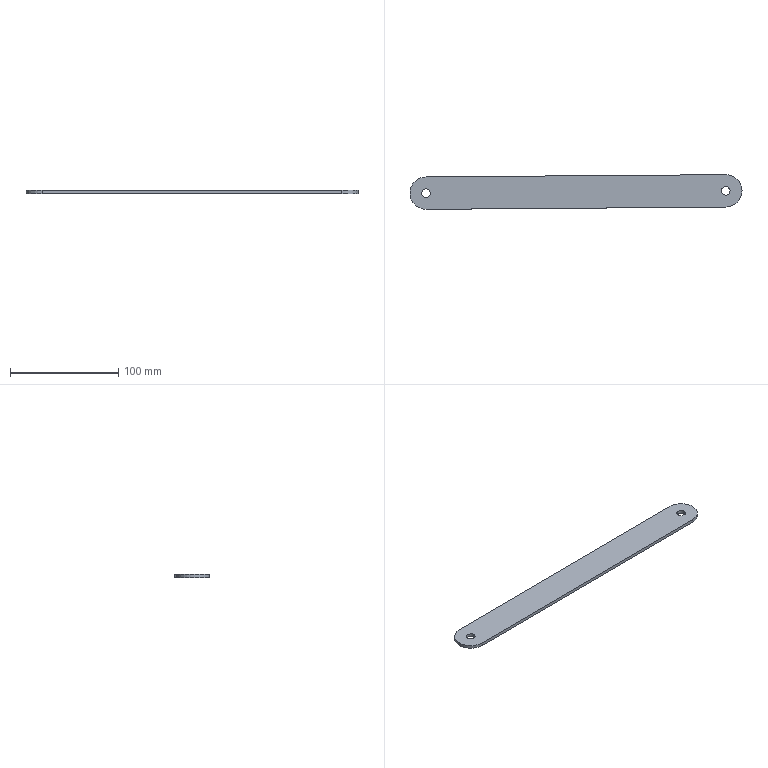Component | SolidWorks | I KOL-1 | 1 solid | 11 faces | box 306.99 x 32.04 x 3 mm | volume 26749 mm3 | cylinder 7 | plane 4 | commonest cylinder face diameters 8 x4 30 x3
STEP:
#1=COLOUR_RGB('',0.7922,0.8196,0.9333);
#2=FILL_AREA_STYLE_COLOUR('',#1);
#3=FILL_AREA_STYLE('',(#2));
#4=SURFACE_STYLE_FILL_AREA(#3);
#5=SURFACE_SIDE_STYLE('',(#4));
#6=SURFACE_STYLE_USAGE(.BOTH.,#5);
#7=PRESENTATION_STYLE_ASSIGNMENT((#6));
#8=CARTESIAN_POINT('',(4.981,6.765,-14.371));
#9=VERTEX_POINT('',#8);
#10=CARTESIAN_POINT('',(5.296,6.767,-14.371));
#11=VERTEX_POINT('',#10);
#12=CARTESIAN_POINT('',(5.139,6.766,-14.371));
#13=DIRECTION('',(0.,0.,1.));
#14=DIRECTION('',(1.,0.007379,0.));
#15=AXIS2_PLACEMENT_3D('',#12,#13,#14);
#16=CIRCLE('',#15,0.1575);
#17=EDGE_CURVE('',#9,#11,#16,.T.);
#18=ORIENTED_EDGE('',*,*,#17,.F.);
#19=CARTESIAN_POINT('',(4.981,6.765,-14.253));
#20=VERTEX_POINT('',#19);
#21=CARTESIAN_POINT('',(4.981,6.765,-14.371));
#22=DIRECTION('',(0.,0.,1.));
#23=VECTOR('',#22,39.37);
#24=LINE('',#21,#23);
#25=EDGE_CURVE('',#9,#20,#24,.T.);
#26=ORIENTED_EDGE('',*,*,#25,.T.);
#27=CARTESIAN_POINT('',(5.296,6.767,-14.253));
#28=VERTEX_POINT('',#27);
#29=CARTESIAN_POINT('',(5.139,6.766,-14.253));
#30=DIRECTION('',(0.,0.,1.));
#31=DIRECTION('',(1.,0.007379,0.));
#32=AXIS2_PLACEMENT_3D('',#29,#30,#31);
#33=CIRCLE('',#32,0.1575);
#34=EDGE_CURVE('',#20,#28,#33,.T.);
#35=ORIENTED_EDGE('',*,*,#34,.T.);
#36=CARTESIAN_POINT('',(5.296,6.767,-14.371));
#37=DIRECTION('',(0.,0.,1.));
#38=VECTOR('',#37,39.37);
#39=LINE('',#36,#38);
#40=EDGE_CURVE('',#11,#28,#39,.T.);
#41=ORIENTED_EDGE('',*,*,#40,.F.);
#42=EDGE_LOOP('',(#18,#26,#35,#41));
#43=FACE_OUTER_BOUND('',#42,.T.);
#44=CARTESIAN_POINT('',(5.139,6.766,-14.371));
#45=DIRECTION('',(0.,0.,1.));
#46=DIRECTION('',(1.,0.007379,0.));
#47=AXIS2_PLACEMENT_3D('',#44,#45,#46);
#48=CYLINDRICAL_SURFACE('',#47,0.1575);
#49=ADVANCED_FACE('',(#43),#48,.F.);
#50=CARTESIAN_POINT('',(-5.924,6.684,-14.371));
#51=VERTEX_POINT('',#50);
#52=CARTESIAN_POINT('',(-5.609,6.686,-14.371));
#53=VERTEX_POINT('',#52);
#54=CARTESIAN_POINT('',(-5.767,6.685,-14.371));
#55=DIRECTION('',(0.,0.,1.));
#56=DIRECTION('',(1.,0.007379,0.));
#57=AXIS2_PLACEMENT_3D('',#54,#55,#56);
#58=CIRCLE('',#57,0.1575);
#59=EDGE_CURVE('',#51,#53,#58,.T.);
#60=ORIENTED_EDGE('',*,*,#59,.F.);
#61=CARTESIAN_POINT('',(-5.924,6.684,-14.253));
#62=VERTEX_POINT('',#61);
#63=CARTESIAN_POINT('',(-5.924,6.684,-14.371));
#64=DIRECTION('',(0.,0.,1.));
#65=VECTOR('',#64,39.37);
#66=LINE('',#63,#65);
#67=EDGE_CURVE('',#51,#62,#66,.T.);
#68=ORIENTED_EDGE('',*,*,#67,.T.);
#69=CARTESIAN_POINT('',(-5.609,6.686,-14.253));
#70=VERTEX_POINT('',#69);
#71=CARTESIAN_POINT('',(-5.767,6.685,-14.253));
#72=DIRECTION('',(0.,0.,1.));
#73=DIRECTION('',(1.,0.007379,0.));
#74=AXIS2_PLACEMENT_3D('',#71,#72,#73);
#75=CIRCLE('',#74,0.1575);
#76=EDGE_CURVE('',#62,#70,#75,.T.);
#77=ORIENTED_EDGE('',*,*,#76,.T.);
#78=CARTESIAN_POINT('',(-5.609,6.686,-14.371));
#79=DIRECTION('',(0.,0.,1.));
#80=VECTOR('',#79,39.37);
#81=LINE('',#78,#80);
#82=EDGE_CURVE('',#53,#70,#81,.T.);
#83=ORIENTED_EDGE('',*,*,#82,.F.);
#84=EDGE_LOOP('',(#60,#68,#77,#83));
#85=FACE_OUTER_BOUND('',#84,.T.);
#86=CARTESIAN_POINT('',(-5.767,6.685,-14.371));
#87=DIRECTION('',(0.,0.,1.));
#88=DIRECTION('',(1.,0.007379,0.));
#89=AXIS2_PLACEMENT_3D('',#86,#87,#88);
#90=CYLINDRICAL_SURFACE('',#89,0.1575);
#91=ADVANCED_FACE('',(#85),#90,.F.);
#92=CARTESIAN_POINT('',(5.143,6.175,-14.371));
#93=VERTEX_POINT('',#92);
#94=CARTESIAN_POINT('',(5.729,6.77,-14.371));
#95=VERTEX_POINT('',#94);
#96=CARTESIAN_POINT('',(5.139,6.766,-14.371));
#97=DIRECTION('',(0.,0.,1.));
#98=DIRECTION('',(1.,0.007379,0.));
#99=AXIS2_PLACEMENT_3D('',#96,#97,#98);
#100=CIRCLE('',#99,0.5906);
#101=EDGE_CURVE('',#93,#95,#100,.T.);
#102=ORIENTED_EDGE('',*,*,#101,.T.);
#103=CARTESIAN_POINT('',(5.729,6.77,-14.253));
#104=VERTEX_POINT('',#103);
#105=CARTESIAN_POINT('',(5.729,6.77,-14.371));
#106=DIRECTION('',(0.,0.,1.));
#107=VECTOR('',#106,39.37);
#108=LINE('',#105,#107);
#109=EDGE_CURVE('',#95,#104,#108,.T.);
#110=ORIENTED_EDGE('',*,*,#109,.T.);
#111=CARTESIAN_POINT('',(5.143,6.175,-14.253));
#112=VERTEX_POINT('',#111);
#113=CARTESIAN_POINT('',(5.139,6.766,-14.253));
#114=DIRECTION('',(0.,0.,1.));
#115=DIRECTION('',(1.,0.007379,0.));
#116=AXIS2_PLACEMENT_3D('',#113,#114,#115);
#117=CIRCLE('',#116,0.5906);
#118=EDGE_CURVE('',#112,#104,#117,.T.);
#119=ORIENTED_EDGE('',*,*,#118,.F.);
#120=CARTESIAN_POINT('',(5.143,6.175,-14.371));
#121=DIRECTION('',(0.,0.,1.));
#122=VECTOR('',#121,39.37);
#123=LINE('',#120,#122);
#124=EDGE_CURVE('',#93,#112,#123,.T.);
#125=ORIENTED_EDGE('',*,*,#124,.F.);
#126=EDGE_LOOP('',(#102,#110,#119,#125));
#127=FACE_OUTER_BOUND('',#126,.T.);
#128=CARTESIAN_POINT('',(5.139,6.766,-14.371));
#129=DIRECTION('',(0.,0.,1.));
#130=DIRECTION('',(1.,0.007379,0.));
#131=AXIS2_PLACEMENT_3D('',#128,#129,#130);
#132=CYLINDRICAL_SURFACE('',#131,0.5906);
#133=ADVANCED_FACE('',(#127),#132,.T.);
#134=CARTESIAN_POINT('',(-5.771,7.276,-14.253));
#135=VERTEX_POINT('',#134);
#136=CARTESIAN_POINT('',(-5.762,6.095,-14.253));
#137=VERTEX_POINT('',#136);
#138=CARTESIAN_POINT('',(-5.767,6.685,-14.253));
#139=DIRECTION('',(0.,0.,1.));
#140=DIRECTION('',(1.,0.007379,0.));
#141=AXIS2_PLACEMENT_3D('',#138,#139,#140);
#142=CIRCLE('',#141,0.5906);
#143=EDGE_CURVE('',#135,#137,#142,.T.);
#144=ORIENTED_EDGE('',*,*,#143,.F.);
#145=CARTESIAN_POINT('',(-5.771,7.276,-14.371));
#146=VERTEX_POINT('',#145);
#147=CARTESIAN_POINT('',(-5.771,7.276,-14.371));
#148=DIRECTION('',(0.,0.,1.));
#149=VECTOR('',#148,39.37);
#150=LINE('',#147,#149);
#151=EDGE_CURVE('',#146,#135,#150,.T.);
#152=ORIENTED_EDGE('',*,*,#151,.F.);
#153=CARTESIAN_POINT('',(-5.762,6.095,-14.371));
#154=VERTEX_POINT('',#153);
#155=CARTESIAN_POINT('',(-5.767,6.685,-14.371));
#156=DIRECTION('',(0.,0.,1.));
#157=DIRECTION('',(1.,0.007379,0.));
#158=AXIS2_PLACEMENT_3D('',#155,#156,#157);
#159=CIRCLE('',#158,0.5906);
#160=EDGE_CURVE('',#146,#154,#159,.T.);
#161=ORIENTED_EDGE('',*,*,#160,.T.);
#162=CARTESIAN_POINT('',(-5.762,6.095,-14.371));
#163=DIRECTION('',(0.,0.,1.));
#164=VECTOR('',#163,39.37);
#165=LINE('',#162,#164);
#166=EDGE_CURVE('',#154,#137,#165,.T.);
#167=ORIENTED_EDGE('',*,*,#166,.T.);
#168=EDGE_LOOP('',(#144,#152,#161,#167));
#169=FACE_OUTER_BOUND('',#168,.T.);
#170=CARTESIAN_POINT('',(-5.767,6.685,-14.371));
#171=DIRECTION('',(0.,0.,1.));
#172=DIRECTION('',(1.,0.007379,0.));
#173=AXIS2_PLACEMENT_3D('',#170,#171,#172);
#174=CYLINDRICAL_SURFACE('',#173,0.5906);
#175=ADVANCED_FACE('',(#169),#174,.T.);
#176=CARTESIAN_POINT('',(5.134,7.356,-14.253));
#177=VERTEX_POINT('',#176);
#178=CARTESIAN_POINT('',(-5.771,7.276,-14.253));
#179=DIRECTION('',(-1.,-0.007379,0.));
#180=VECTOR('',#179,39.37);
#181=LINE('',#178,#180);
#182=EDGE_CURVE('',#177,#135,#181,.T.);
#183=ORIENTED_EDGE('',*,*,#182,.F.);
#184=CARTESIAN_POINT('',(5.134,7.356,-14.371));
#185=VERTEX_POINT('',#184);
#186=CARTESIAN_POINT('',(5.134,7.356,-14.371));
#187=DIRECTION('',(0.,0.,1.));
#188=VECTOR('',#187,39.37);
#189=LINE('',#186,#188);
#190=EDGE_CURVE('',#185,#177,#189,.T.);
#191=ORIENTED_EDGE('',*,*,#190,.F.);
#192=CARTESIAN_POINT('',(-5.771,7.276,-14.371));
#193=DIRECTION('',(-1.,-0.007379,0.));
#194=VECTOR('',#193,39.37);
#195=LINE('',#192,#194);
#196=EDGE_CURVE('',#185,#146,#195,.T.);
#197=ORIENTED_EDGE('',*,*,#196,.T.);
#198=ORIENTED_EDGE('',*,*,#151,.T.);
#199=EDGE_LOOP('',(#183,#191,#197,#198));
#200=FACE_OUTER_BOUND('',#199,.T.);
#201=CARTESIAN_POINT('',(-5.771,7.276,-14.371));
#202=DIRECTION('',(-0.007379,1.,-0.));
#203=DIRECTION('',(0.,0.,1.));
#204=AXIS2_PLACEMENT_3D('',#201,#202,#203);
#205=PLANE('',#204);
#206=ADVANCED_FACE('',(#200),#205,.T.);
#207=ORIENTED_EDGE('',*,*,#109,.F.);
#208=CARTESIAN_POINT('',(5.139,6.766,-14.371));
#209=DIRECTION('',(0.,0.,1.));
#210=DIRECTION('',(1.,0.007379,0.));
#211=AXIS2_PLACEMENT_3D('',#208,#209,#210);
#212=CIRCLE('',#211,0.5906);
#213=EDGE_CURVE('',#95,#185,#212,.T.);
#214=ORIENTED_EDGE('',*,*,#213,.T.);
#215=ORIENTED_EDGE('',*,*,#190,.T.);
#216=CARTESIAN_POINT('',(5.139,6.766,-14.253));
#217=DIRECTION('',(0.,0.,1.));
#218=DIRECTION('',(1.,0.007379,0.));
#219=AXIS2_PLACEMENT_3D('',#216,#217,#218);
#220=CIRCLE('',#219,0.5906);
#221=EDGE_CURVE('',#104,#177,#220,.T.);
#222=ORIENTED_EDGE('',*,*,#221,.F.);
#223=EDGE_LOOP('',(#207,#214,#215,#222));
#224=FACE_OUTER_BOUND('',#223,.T.);
#225=CARTESIAN_POINT('',(5.139,6.766,-14.371));
#226=DIRECTION('',(0.,0.,1.));
#227=DIRECTION('',(1.,0.007379,0.));
#228=AXIS2_PLACEMENT_3D('',#225,#226,#227);
#229=CYLINDRICAL_SURFACE('',#228,0.5906);
#230=ADVANCED_FACE('',(#224),#229,.T.);
#231=CARTESIAN_POINT('',(-5.762,6.095,-14.253));
#232=DIRECTION('',(1.,0.007379,-0.));
#233=VECTOR('',#232,39.37);
#234=LINE('',#231,#233);
#235=EDGE_CURVE('',#137,#112,#234,.T.);
#236=ORIENTED_EDGE('',*,*,#235,.F.);
#237=ORIENTED_EDGE('',*,*,#166,.F.);
#238=CARTESIAN_POINT('',(-5.762,6.095,-14.371));
#239=DIRECTION('',(1.,0.007379,-0.));
#240=VECTOR('',#239,39.37);
#241=LINE('',#238,#240);
#242=EDGE_CURVE('',#154,#93,#241,.T.);
#243=ORIENTED_EDGE('',*,*,#242,.T.);
#244=ORIENTED_EDGE('',*,*,#124,.T.);
#245=EDGE_LOOP('',(#236,#237,#243,#244));
#246=FACE_OUTER_BOUND('',#245,.T.);
#247=CARTESIAN_POINT('',(-5.762,6.095,-14.371));
#248=DIRECTION('',(0.007379,-1.,0.));
#249=DIRECTION('',(-0.,-0.,-1.));
#250=AXIS2_PLACEMENT_3D('',#247,#248,#249);
#251=PLANE('',#250);
#252=ADVANCED_FACE('',(#246),#251,.T.);
#253=CARTESIAN_POINT('',(5.139,6.766,-14.371));
#254=DIRECTION('',(0.,0.,1.));
#255=DIRECTION('',(1.,0.007379,0.));
#256=AXIS2_PLACEMENT_3D('',#253,#254,#255);
#257=CIRCLE('',#256,0.1575);
#258=EDGE_CURVE('',#11,#9,#257,.T.);
#259=ORIENTED_EDGE('',*,*,#258,.T.);
#260=ORIENTED_EDGE('',*,*,#17,.T.);
#261=EDGE_LOOP('',(#259,#260));
#262=FACE_BOUND('',#261,.T.);
#263=CARTESIAN_POINT('',(-5.767,6.685,-14.371));
#264=DIRECTION('',(0.,0.,1.));
#265=DIRECTION('',(1.,0.007379,0.));
#266=AXIS2_PLACEMENT_3D('',#263,#264,#265);
#267=CIRCLE('',#266,0.1575);
#268=EDGE_CURVE('',#53,#51,#267,.T.);
#269=ORIENTED_EDGE('',*,*,#268,.T.);
#270=ORIENTED_EDGE('',*,*,#59,.T.);
#271=EDGE_LOOP('',(#269,#270));
#272=FACE_BOUND('',#271,.T.);
#273=ORIENTED_EDGE('',*,*,#160,.F.);
#274=ORIENTED_EDGE('',*,*,#196,.F.);
#275=ORIENTED_EDGE('',*,*,#213,.F.);
#276=ORIENTED_EDGE('',*,*,#101,.F.);
#277=ORIENTED_EDGE('',*,*,#242,.F.);
#278=EDGE_LOOP('',(#273,#274,#275,#276,#277));
#279=FACE_OUTER_BOUND('',#278,.T.);
#280=CARTESIAN_POINT('',(-5.767,6.685,-14.371));
#281=DIRECTION('',(0.,0.,1.));
#282=DIRECTION('',(1.,0.007379,-0.));
#283=AXIS2_PLACEMENT_3D('',#280,#281,#282);
#284=PLANE('',#283);
#285=ADVANCED_FACE('',(#262,#272,#279),#284,.F.);
#286=CARTESIAN_POINT('',(5.139,6.766,-14.253));
#287=DIRECTION('',(0.,0.,1.));
#288=DIRECTION('',(1.,0.007379,0.));
#289=AXIS2_PLACEMENT_3D('',#286,#287,#288);
#290=CIRCLE('',#289,0.1575);
#291=EDGE_CURVE('',#28,#20,#290,.T.);
#292=ORIENTED_EDGE('',*,*,#291,.F.);
#293=ORIENTED_EDGE('',*,*,#34,.F.);
#294=EDGE_LOOP('',(#292,#293));
#295=FACE_BOUND('',#294,.T.);
#296=CARTESIAN_POINT('',(-5.767,6.685,-14.253));
#297=DIRECTION('',(0.,0.,1.));
#298=DIRECTION('',(1.,0.007379,0.));
#299=AXIS2_PLACEMENT_3D('',#296,#297,#298);
#300=CIRCLE('',#299,0.1575);
#301=EDGE_CURVE('',#70,#62,#300,.T.);
#302=ORIENTED_EDGE('',*,*,#301,.F.);
#303=ORIENTED_EDGE('',*,*,#76,.F.);
#304=EDGE_LOOP('',(#302,#303));
#305=FACE_BOUND('',#304,.T.);
#306=ORIENTED_EDGE('',*,*,#143,.T.);
#307=ORIENTED_EDGE('',*,*,#235,.T.);
#308=ORIENTED_EDGE('',*,*,#118,.T.);
#309=ORIENTED_EDGE('',*,*,#221,.T.);
#310=ORIENTED_EDGE('',*,*,#182,.T.);
#311=EDGE_LOOP('',(#306,#307,#308,#309,#310));
#312=FACE_OUTER_BOUND('',#311,.T.);
#313=CARTESIAN_POINT('',(-5.767,6.685,-14.253));
#314=DIRECTION('',(0.,0.,1.));
#315=DIRECTION('',(1.,0.007379,-0.));
#316=AXIS2_PLACEMENT_3D('',#313,#314,#315);
#317=PLANE('',#316);
#318=ADVANCED_FACE('',(#295,#305,#312),#317,.T.);
#319=ORIENTED_EDGE('',*,*,#67,.F.);
#320=ORIENTED_EDGE('',*,*,#268,.F.);
#321=ORIENTED_EDGE('',*,*,#82,.T.);
#322=ORIENTED_EDGE('',*,*,#301,.T.);
#323=EDGE_LOOP('',(#319,#320,#321,#322));
#324=FACE_OUTER_BOUND('',#323,.T.);
#325=CARTESIAN_POINT('',(-5.767,6.685,-14.371));
#326=DIRECTION('',(0.,0.,1.));
#327=DIRECTION('',(1.,0.007379,0.));
#328=AXIS2_PLACEMENT_3D('',#325,#326,#327);
#329=CYLINDRICAL_SURFACE('',#328,0.1575);
#330=ADVANCED_FACE('',(#324),#329,.F.);
#331=ORIENTED_EDGE('',*,*,#25,.F.);
#332=ORIENTED_EDGE('',*,*,#258,.F.);
#333=ORIENTED_EDGE('',*,*,#40,.T.);
#334=ORIENTED_EDGE('',*,*,#291,.T.);
#335=EDGE_LOOP('',(#331,#332,#333,#334));
#336=FACE_OUTER_BOUND('',#335,.T.);
#337=CARTESIAN_POINT('',(5.139,6.766,-14.371));
#338=DIRECTION('',(0.,0.,1.));
#339=DIRECTION('',(1.,0.007379,0.));
#340=AXIS2_PLACEMENT_3D('',#337,#338,#339);
#341=CYLINDRICAL_SURFACE('',#340,0.1575);
#342=ADVANCED_FACE('',(#336),#341,.F.);
#343=CLOSED_SHELL('',(#49,#91,#133,#175,#206,#230,#252,#285,#318,#330,#342));
#344=MANIFOLD_SOLID_BREP('',#343);
#345=STYLED_ITEM('',(#7),#344);
#346=(LENGTH_UNIT()NAMED_UNIT(*)SI_UNIT($,.METRE.));
#347=LENGTH_MEASURE_WITH_UNIT(LENGTH_MEASURE(0.0254),#346);
#348=DIMENSIONAL_EXPONENTS(1.,0.,0.,0.,0.,0.,0.);
#349=(CONVERSION_BASED_UNIT('',#347)LENGTH_UNIT()NAMED_UNIT(#348));
#350=UNCERTAINTY_MEASURE_WITH_UNIT(LENGTH_MEASURE(0.00001),#349,'','');
#351=(NAMED_UNIT(*)PLANE_ANGLE_UNIT()SI_UNIT($,.RADIAN.));
#352=(NAMED_UNIT(*)SI_UNIT($,.STERADIAN.)SOLID_ANGLE_UNIT());
#353=(GEOMETRIC_REPRESENTATION_CONTEXT(3)GLOBAL_UNCERTAINTY_ASSIGNED_CONTEXT((#350))GLOBAL_UNIT_ASSIGNED_CONTEXT((#349,#351,#352))REPRESENTATION_CONTEXT('',''));
#354=MECHANICAL_DESIGN_GEOMETRIC_PRESENTATION_REPRESENTATION('',(#345),#353);
#355=CARTESIAN_POINT('',(0.,0.,0.));
#356=DIRECTION('',(0.,0.,1.));
#357=DIRECTION('',(1.,0.,0.));
#358=AXIS2_PLACEMENT_3D('',#355,#356,#357);
#359=(LENGTH_UNIT()NAMED_UNIT(*)SI_UNIT($,.METRE.));
#360=LENGTH_MEASURE_WITH_UNIT(LENGTH_MEASURE(0.0254),#359);
#361=DIMENSIONAL_EXPONENTS(1.,0.,0.,0.,0.,0.,0.);
#362=(CONVERSION_BASED_UNIT('',#360)LENGTH_UNIT()NAMED_UNIT(#361));
#363=UNCERTAINTY_MEASURE_WITH_UNIT(LENGTH_MEASURE(0.00001),#362,'','');
#364=(NAMED_UNIT(*)PLANE_ANGLE_UNIT()SI_UNIT($,.RADIAN.));
#365=(NAMED_UNIT(*)SI_UNIT($,.STERADIAN.)SOLID_ANGLE_UNIT());
#366=(GEOMETRIC_REPRESENTATION_CONTEXT(3)GLOBAL_UNCERTAINTY_ASSIGNED_CONTEXT((#363))GLOBAL_UNIT_ASSIGNED_CONTEXT((#362,#364,#365))REPRESENTATION_CONTEXT('',''));
#367=ADVANCED_BREP_SHAPE_REPRESENTATION('',(#344,#358),#366);
#368=PRESENTATION_LAYER_ASSIGNMENT('','',(#345));